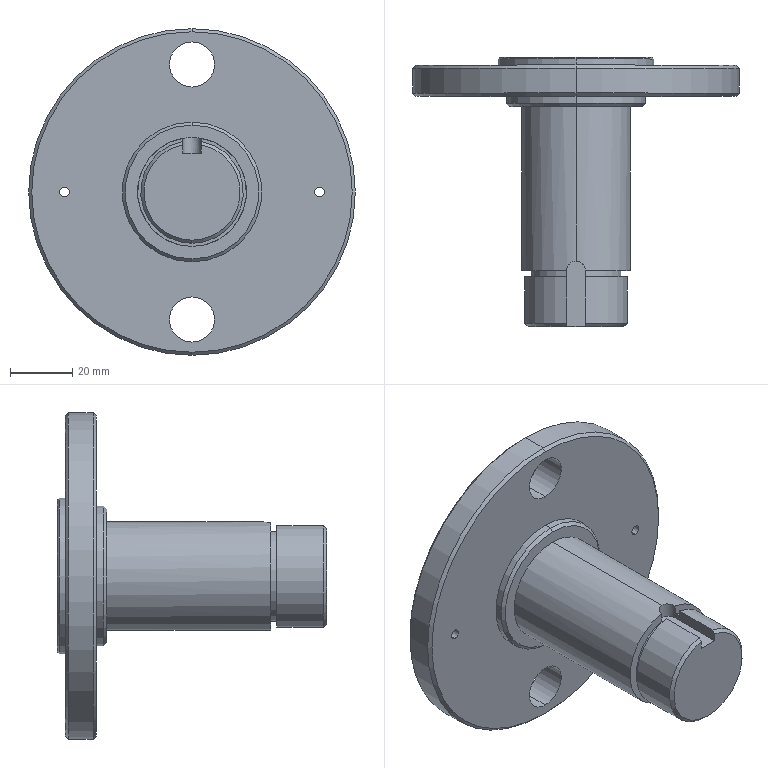Component | SolidWorks | MA060.03.03-04-1 | 1 solid | 50 faces | volume 155815 mm3 | cylinder 26 | cone 12 | plane 12 | commonest cylinder face diameters 6 x5 3.2 x4 14.5 x4 10 x2 50 x2 105 x2 45 x2 29 x2 | material 45#